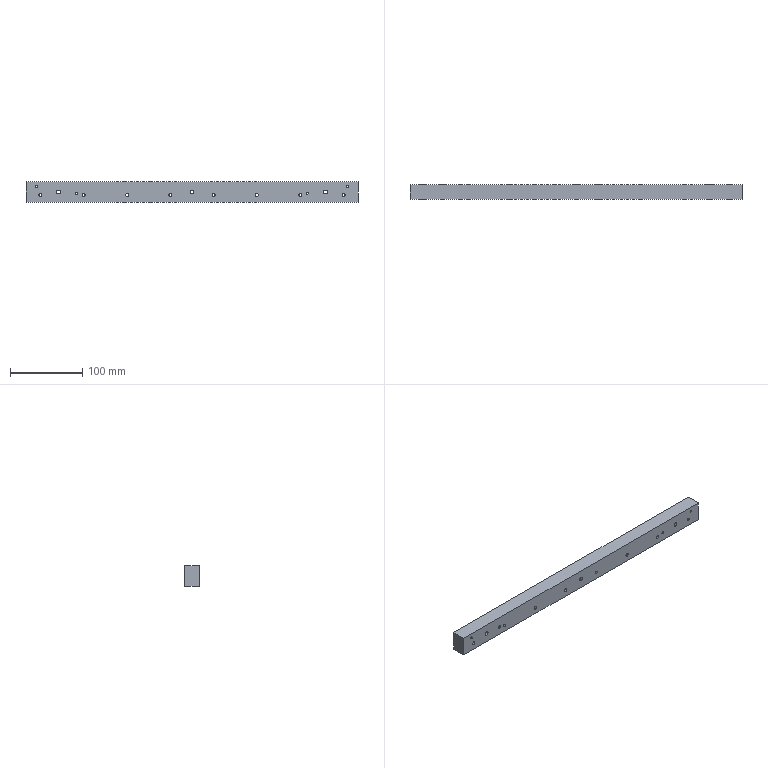Component | SolidWorks | SFTJ-05-GuidePlate-1 | 1 solid | 47 faces | box 460 x 20 x 28 mm | volume 252498 mm3 | cylinder 36 | plane 11 | commonest cylinder face diameters 4.2 x16 3 x8 10 x6 5.3 x6 | material 6061 Alloy
build123d program:
from build123d import *

# Parameters (mm, degrees)
SKETCH1_W                                            = 28
SKETCH1_H                                            = 460
BOSS_EXTRUDE1_DEPTH                                  = 10
SIZE_MM_DOWEL_PIN_HOLE2_D                            = 3
CUT_EXTRUDE1_DEPTH                                   = 232.292
SIZE_MM_DOWEL_PIN_HOLE2_2_D                          = 3
M5_TAPPED_HOLE1_D                                    = 4.2
HOLE_SIZE_ACCORDING_TO_HEX_SOCKET_HEAD_C_D           = 5.3
HOLE_SIZE_ACCORDING_TO_HEX_SOCKET_HEAD_C_CBORE_D     = 10
HOLE_SIZE_ACCORDING_TO_HEX_SOCKET_HEAD_C_CBORE_DEPTH = 5.7


with BuildPart() as part:
    # Sketch1 → Boss-Extrude1 (new, symmetric)
    with BuildSketch(Plane.XY):
        Rectangle(SKETCH1_W, SKETCH1_H)
    extrude(amount=BOSS_EXTRUDE1_DEPTH, both=True)

    # Size mm Dowel Pin Hole2 (through all)
    with Locations(Plane.XY.offset(10)):
        with Locations((1.5, 160)):
            Hole(SIZE_MM_DOWEL_PIN_HOLE2_D / 2)

    # Sketch6 → Cut-Extrude1 (cut, through all)
    with BuildSketch(Plane.XY.offset(10)):
        with BuildLine():
            Line((3, -159.75), (3, -160.25))
            ThreePointArc((3, -160.25), (1.5, -161.75), (0, -160.25))
            Line((0, -160.25), (0, -159.75))
            ThreePointArc((0, -159.75), (1.5, -158.25), (3, -159.75))
        make_face()
    extrude(amount=-CUT_EXTRUDE1_DEPTH, mode=Mode.SUBTRACT)

    # Size mm Dowel Pin Hole2_2 (through all)
    with Locations(Plane(origin=(0, 0, -10), x_dir=(-1, 0, 0), z_dir=(0, 0, -1))):
        with Locations((7.5, -215), (7.5, 215)):
            Hole(SIZE_MM_DOWEL_PIN_HOLE2_2_D / 2)

    # M5 Tapped Hole1 (through all)
    with Locations(Plane(origin=(0, 0, -10), x_dir=(-1, 0, 0), z_dir=(0, 0, -1))):
        with Locations((-4, -210), (-4, -150), (-4, -90), (-4, -30), (-4, 30), (-4, 90), (-4, 150), (-4, 210)):
            Hole(M5_TAPPED_HOLE1_D / 2)

    # Hole Size according to Hex Socket Head C (through all)
    with Locations(Plane(origin=(0, 0, -10), x_dir=(-1, 0, 0), z_dir=(0, 0, -1))):
        with Locations((0, 185), (0, 0), (0, -185)):
            CounterBoreHole(HOLE_SIZE_ACCORDING_TO_HEX_SOCKET_HEAD_C_D / 2, HOLE_SIZE_ACCORDING_TO_HEX_SOCKET_HEAD_C_CBORE_D / 2, HOLE_SIZE_ACCORDING_TO_HEX_SOCKET_HEAD_C_CBORE_DEPTH)


solid = part.part

# Placed as in the assembly
solid = solid.moved(Location((-97.009, 2.721, 98.589), (90, 0, -90)))